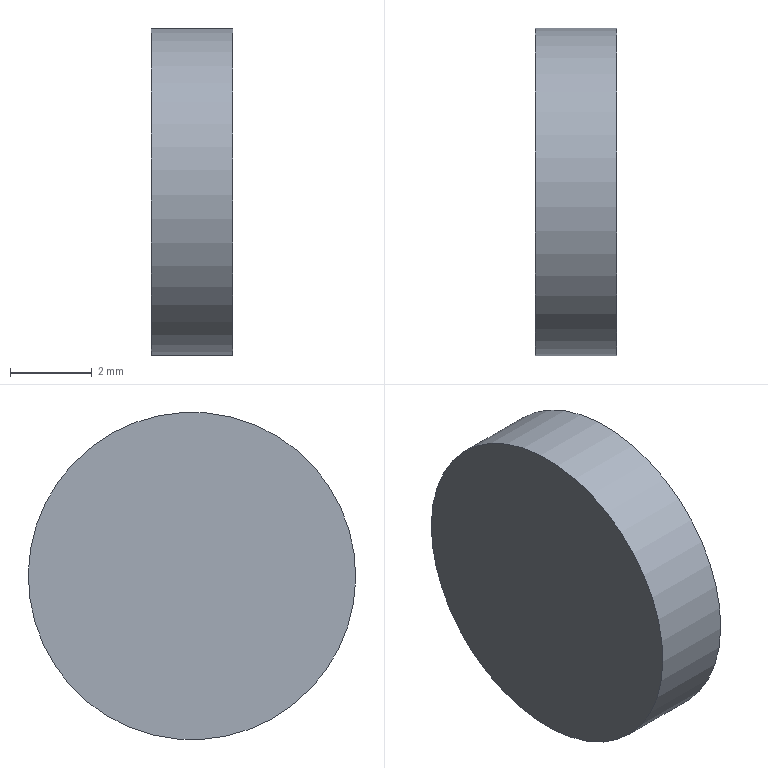Component | NX | BUTTONA_2 | 1 solid | 3 faces | box 2 x 8 x 8 mm | volume 101 mm3 | plane 2 | cylinder 1 | commonest cylinder face diameters 8 x1
STEP:
#1=CARTESIAN_POINT('',(0.,0.,0.));
#2=DIRECTION('',(0.,0.,1.));
#3=DIRECTION('',(1.,0.,0.));
#4=AXIS2_PLACEMENT_3D('',#1,#2,#3);
#5=CARTESIAN_POINT('',(-108.42,163.73,20.169));
#6=VERTEX_POINT('',#5);
#7=CARTESIAN_POINT('',(-108.42,165.257,16.472));
#8=DIRECTION('',(-1.,0.,0.));
#9=DIRECTION('',(0.,-0.3818,0.9242));
#10=AXIS2_PLACEMENT_3D('',#7,#8,#9);
#11=CIRCLE('',#10,4.);
#12=CARTESIAN_POINT('',(-108.42,165.257,16.472));
#13=DIRECTION('',(1.,0.,0.));
#14=DIRECTION('',(0.,0.9242,0.3818));
#15=AXIS2_PLACEMENT_3D('',#12,#13,#14);
#16=PLANE('',#15);
#17=CARTESIAN_POINT('',(-0.,4.));
#18=CARTESIAN_POINT('',(6.928,4.));
#19=CARTESIAN_POINT('',(3.464,-2.));
#20=CARTESIAN_POINT('',(0.,-8.));
#21=CARTESIAN_POINT('',(-3.464,-2.));
#22=CARTESIAN_POINT('',(-6.928,4.));
#23=CARTESIAN_POINT('',(-0.,4.));
#24=(BOUNDED_CURVE()B_SPLINE_CURVE(2,(#17,#18,#19,#20,#21,#22,#23),.UNSPECIFIED.,.T.,.F.)B_SPLINE_CURVE_WITH_KNOTS((1,2,2,2,2,1),(-2.094,0.,2.094,4.189,6.283,8.378),.UNSPECIFIED.)CURVE()GEOMETRIC_REPRESENTATION_ITEM()RATIONAL_B_SPLINE_CURVE((1.,0.5,1.,0.5,1.,0.5,1.))REPRESENTATION_ITEM(''));
#25=(GEOMETRIC_REPRESENTATION_CONTEXT(2)PARAMETRIC_REPRESENTATION_CONTEXT()REPRESENTATION_CONTEXT('',''));
#26=DEFINITIONAL_REPRESENTATION('',(#24),#25);
#27=PCURVE('',#16,#26);
#28=CARTESIAN_POINT('',(-110.42,165.257,16.472));
#29=DIRECTION('',(1.,0.,0.));
#30=DIRECTION('',(0.,-0.3818,0.9242));
#31=AXIS2_PLACEMENT_3D('',#28,#29,#30);
#32=CYLINDRICAL_SURFACE('',#31,4.);
#33=CARTESIAN_POINT('',(6.283,2.));
#34=DIRECTION('',(-1.,0.));
#35=VECTOR('',#34,1.);
#36=LINE('',#33,#35);
#37=(GEOMETRIC_REPRESENTATION_CONTEXT(2)PARAMETRIC_REPRESENTATION_CONTEXT()REPRESENTATION_CONTEXT('',''));
#38=DEFINITIONAL_REPRESENTATION('',(#36),#37);
#39=PCURVE('',#32,#38);
#40=SURFACE_CURVE('',#11,(#27,#39),.PCURVE_S1.);
#41=EDGE_CURVE('',#6,#6,#40,.T.);
#42=ORIENTED_EDGE('',*,*,#41,.F.);
#43=EDGE_LOOP('',(#42));
#44=FACE_BOUND('',#43,.T.);
#45=ADVANCED_FACE('',(#44),#16,.T.);
#46=CARTESIAN_POINT('',(-110.42,163.73,20.169));
#47=VERTEX_POINT('',#46);
#48=CARTESIAN_POINT('',(-110.42,165.257,16.472));
#49=DIRECTION('',(1.,0.,0.));
#50=DIRECTION('',(0.,-0.3818,0.9242));
#51=AXIS2_PLACEMENT_3D('',#48,#49,#50);
#52=CIRCLE('',#51,4.);
#53=CARTESIAN_POINT('',(-110.42,165.257,16.472));
#54=DIRECTION('',(-1.,0.,0.));
#55=DIRECTION('',(0.,-0.9242,-0.3818));
#56=AXIS2_PLACEMENT_3D('',#53,#54,#55);
#57=PLANE('',#56);
#58=CARTESIAN_POINT('',(0.,4.));
#59=CARTESIAN_POINT('',(6.928,4.));
#60=CARTESIAN_POINT('',(3.464,-2.));
#61=CARTESIAN_POINT('',(-0.,-8.));
#62=CARTESIAN_POINT('',(-3.464,-2.));
#63=CARTESIAN_POINT('',(-6.928,4.));
#64=CARTESIAN_POINT('',(0.,4.));
#65=(BOUNDED_CURVE()B_SPLINE_CURVE(2,(#58,#59,#60,#61,#62,#63,#64),.UNSPECIFIED.,.T.,.F.)B_SPLINE_CURVE_WITH_KNOTS((1,2,2,2,2,1),(-2.094,0.,2.094,4.189,6.283,8.378),.UNSPECIFIED.)CURVE()GEOMETRIC_REPRESENTATION_ITEM()RATIONAL_B_SPLINE_CURVE((1.,0.5,1.,0.5,1.,0.5,1.))REPRESENTATION_ITEM(''));
#66=(GEOMETRIC_REPRESENTATION_CONTEXT(2)PARAMETRIC_REPRESENTATION_CONTEXT()REPRESENTATION_CONTEXT('',''));
#67=DEFINITIONAL_REPRESENTATION('',(#65),#66);
#68=PCURVE('',#57,#67);
#69=CARTESIAN_POINT('',(0.,0.));
#70=DIRECTION('',(1.,0.));
#71=VECTOR('',#70,1.);
#72=LINE('',#69,#71);
#73=(GEOMETRIC_REPRESENTATION_CONTEXT(2)PARAMETRIC_REPRESENTATION_CONTEXT()REPRESENTATION_CONTEXT('',''));
#74=DEFINITIONAL_REPRESENTATION('',(#72),#73);
#75=PCURVE('',#32,#74);
#76=SURFACE_CURVE('',#52,(#68,#75),.PCURVE_S1.);
#77=EDGE_CURVE('',#47,#47,#76,.T.);
#78=ORIENTED_EDGE('',*,*,#77,.F.);
#79=EDGE_LOOP('',(#78));
#80=FACE_BOUND('',#79,.T.);
#81=ADVANCED_FACE('',(#80),#57,.T.);
#82=ORIENTED_EDGE('',*,*,#41,.T.);
#83=CARTESIAN_POINT('',(-110.42,163.73,20.169));
#84=CARTESIAN_POINT('',(-108.42,163.73,20.169));
#85=B_SPLINE_CURVE_WITH_KNOTS('',1,(#83,#84),.UNSPECIFIED.,.F.,.F.,(2,2),(0.,2.),.PIECEWISE_BEZIER_KNOTS.);
#86=CARTESIAN_POINT('',(0.,0.));
#87=DIRECTION('',(0.,1.));
#88=VECTOR('',#87,1.);
#89=LINE('',#86,#88);
#90=(GEOMETRIC_REPRESENTATION_CONTEXT(2)PARAMETRIC_REPRESENTATION_CONTEXT()REPRESENTATION_CONTEXT('',''));
#91=DEFINITIONAL_REPRESENTATION('',(#89),#90);
#92=PCURVE('',#32,#91);
#93=CARTESIAN_POINT('',(6.283,0.));
#94=DIRECTION('',(0.,1.));
#95=VECTOR('',#94,1.);
#96=LINE('',#93,#95);
#97=(GEOMETRIC_REPRESENTATION_CONTEXT(2)PARAMETRIC_REPRESENTATION_CONTEXT()REPRESENTATION_CONTEXT('',''));
#98=DEFINITIONAL_REPRESENTATION('',(#96),#97);
#99=PCURVE('',#32,#98);
#100=SEAM_CURVE('',#85,(#92,#99),.PCURVE_S1.);
#101=EDGE_CURVE('',#47,#6,#100,.T.);
#102=ORIENTED_EDGE('',*,*,#101,.F.);
#103=ORIENTED_EDGE('',*,*,#77,.T.);
#104=ORIENTED_EDGE('',*,*,#101,.T.);
#105=EDGE_LOOP('',(#82,#102,#103,#104));
#106=FACE_BOUND('',#105,.T.);
#107=ADVANCED_FACE('',(#106),#32,.T.);
#108=CLOSED_SHELL('',(#45,#81,#107));
#109=MANIFOLD_SOLID_BREP('',#108);
#110=(LENGTH_UNIT()NAMED_UNIT(*)SI_UNIT(.MILLI.,.METRE.));
#111=UNCERTAINTY_MEASURE_WITH_UNIT(LENGTH_MEASURE(0.00001),#110,'','');
#112=(NAMED_UNIT(*)PLANE_ANGLE_UNIT()SI_UNIT($,.RADIAN.));
#113=(NAMED_UNIT(*)SI_UNIT($,.STERADIAN.)SOLID_ANGLE_UNIT());
#114=(GEOMETRIC_REPRESENTATION_CONTEXT(3)GLOBAL_UNCERTAINTY_ASSIGNED_CONTEXT((#111))GLOBAL_UNIT_ASSIGNED_CONTEXT((#110,#112,#113))REPRESENTATION_CONTEXT('',''));
#115=ADVANCED_BREP_SHAPE_REPRESENTATION('',(#4,#109),#114);